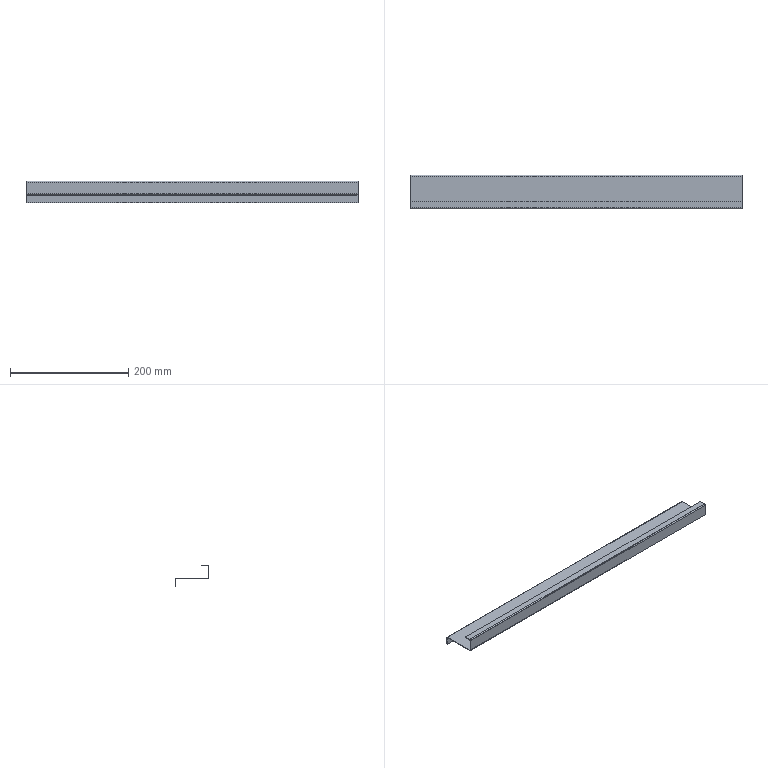Component | SolidWorks | CCQ-1.1-13UpperBeam2-1 | 1 solid | 30 faces | box 561 x 56.74 x 37 mm | volume 57303 mm3 | plane 24 | cylinder 6 | commonest cylinder face diameters 3.473 x3 1.473 x3 | material 304
STEP:
#1=COLOUR_RGB('',0.7922,0.8196,0.9333);
#2=FILL_AREA_STYLE_COLOUR('',#1);
#3=FILL_AREA_STYLE('',(#2));
#4=SURFACE_STYLE_FILL_AREA(#3);
#5=SURFACE_SIDE_STYLE('',(#4));
#6=SURFACE_STYLE_USAGE(.BOTH.,#5);
#7=PRESENTATION_STYLE_ASSIGNMENT((#6));
#8=CARTESIAN_POINT('',(-1.161,26.014,0.8164));
#9=VERTEX_POINT('',#8);
#10=CARTESIAN_POINT('',(-1.161,26.054,0.8164));
#11=VERTEX_POINT('',#10);
#12=CARTESIAN_POINT('',(-1.161,26.014,0.8164));
#13=DIRECTION('',(0.,1.,0.));
#14=VECTOR('',#13,39.37);
#15=LINE('',#12,#14);
#16=EDGE_CURVE('',#9,#11,#15,.T.);
#17=ORIENTED_EDGE('',*,*,#16,.F.);
#18=CARTESIAN_POINT('',(-1.161,26.083,0.748));
#19=VERTEX_POINT('',#18);
#20=CARTESIAN_POINT('',(-1.161,26.083,0.8164));
#21=DIRECTION('',(-1.,0.,0.));
#22=DIRECTION('',(0.,0.,-1.));
#23=AXIS2_PLACEMENT_3D('',#20,#21,#22);
#24=CIRCLE('',#23,0.06837);
#25=EDGE_CURVE('',#19,#9,#24,.T.);
#26=ORIENTED_EDGE('',*,*,#25,.F.);
#27=CARTESIAN_POINT('',(-1.161,26.083,0.7874));
#28=VERTEX_POINT('',#27);
#29=CARTESIAN_POINT('',(-1.161,26.083,0.7874));
#30=DIRECTION('',(0.,0.,-1.));
#31=VECTOR('',#30,39.37);
#32=LINE('',#29,#31);
#33=EDGE_CURVE('',#28,#19,#32,.T.);
#34=ORIENTED_EDGE('',*,*,#33,.F.);
#35=CARTESIAN_POINT('',(-1.161,26.083,0.8164));
#36=DIRECTION('',(-1.,0.,0.));
#37=DIRECTION('',(0.,0.,-1.));
#38=AXIS2_PLACEMENT_3D('',#35,#36,#37);
#39=CIRCLE('',#38,0.029);
#40=EDGE_CURVE('',#28,#11,#39,.T.);
#41=ORIENTED_EDGE('',*,*,#40,.T.);
#42=EDGE_LOOP('',(#17,#26,#34,#41));
#43=FACE_OUTER_BOUND('',#42,.T.);
#44=CARTESIAN_POINT('',(-1.161,26.014,0.8164));
#45=DIRECTION('',(1.,0.,0.));
#46=DIRECTION('',(0.,0.,-1.));
#47=AXIS2_PLACEMENT_3D('',#44,#45,#46);
#48=PLANE('',#47);
#49=ADVANCED_FACE('',(#43),#48,.T.);
#50=CARTESIAN_POINT('',(-1.161,26.014,1.585));
#51=VERTEX_POINT('',#50);
#52=CARTESIAN_POINT('',(-1.161,26.014,0.748));
#53=DIRECTION('',(0.,-0.,1.));
#54=VECTOR('',#53,39.37);
#55=LINE('',#52,#54);
#56=EDGE_CURVE('',#9,#51,#55,.T.);
#57=ORIENTED_EDGE('',*,*,#56,.F.);
#58=ORIENTED_EDGE('',*,*,#16,.T.);
#59=CARTESIAN_POINT('',(-1.161,26.054,1.585));
#60=VERTEX_POINT('',#59);
#61=CARTESIAN_POINT('',(-1.161,26.054,0.748));
#62=DIRECTION('',(0.,-0.,1.));
#63=VECTOR('',#62,39.37);
#64=LINE('',#61,#63);
#65=EDGE_CURVE('',#11,#60,#64,.T.);
#66=ORIENTED_EDGE('',*,*,#65,.T.);
#67=CARTESIAN_POINT('',(-1.161,26.054,1.585));
#68=DIRECTION('',(0.,-1.,0.));
#69=VECTOR('',#68,39.37);
#70=LINE('',#67,#69);
#71=EDGE_CURVE('',#60,#51,#70,.T.);
#72=ORIENTED_EDGE('',*,*,#71,.T.);
#73=EDGE_LOOP('',(#57,#58,#66,#72));
#74=FACE_OUTER_BOUND('',#73,.T.);
#75=CARTESIAN_POINT('',(-1.161,26.083,0.7874));
#76=DIRECTION('',(1.,0.,0.));
#77=DIRECTION('',(0.,0.,-1.));
#78=AXIS2_PLACEMENT_3D('',#75,#76,#77);
#79=PLANE('',#78);
#80=ADVANCED_FACE('',(#74),#79,.T.);
#81=CARTESIAN_POINT('',(-23.248,26.083,0.748));
#82=VERTEX_POINT('',#81);
#83=CARTESIAN_POINT('',(-23.248,26.083,0.7874));
#84=VERTEX_POINT('',#83);
#85=CARTESIAN_POINT('',(-23.248,26.083,0.748));
#86=DIRECTION('',(0.,0.,1.));
#87=VECTOR('',#86,39.37);
#88=LINE('',#85,#87);
#89=EDGE_CURVE('',#82,#84,#88,.T.);
#90=ORIENTED_EDGE('',*,*,#89,.F.);
#91=CARTESIAN_POINT('',(-23.248,26.014,0.8164));
#92=VERTEX_POINT('',#91);
#93=CARTESIAN_POINT('',(-23.248,26.083,0.8164));
#94=DIRECTION('',(-1.,0.,0.));
#95=DIRECTION('',(0.,0.,-1.));
#96=AXIS2_PLACEMENT_3D('',#93,#94,#95);
#97=CIRCLE('',#96,0.06837);
#98=EDGE_CURVE('',#82,#92,#97,.T.);
#99=ORIENTED_EDGE('',*,*,#98,.T.);
#100=CARTESIAN_POINT('',(-23.248,26.054,0.8164));
#101=VERTEX_POINT('',#100);
#102=CARTESIAN_POINT('',(-23.248,26.054,0.8164));
#103=DIRECTION('',(0.,-1.,-0.));
#104=VECTOR('',#103,39.37);
#105=LINE('',#102,#104);
#106=EDGE_CURVE('',#101,#92,#105,.T.);
#107=ORIENTED_EDGE('',*,*,#106,.F.);
#108=CARTESIAN_POINT('',(-23.248,26.083,0.8164));
#109=DIRECTION('',(-1.,0.,0.));
#110=DIRECTION('',(0.,0.,-1.));
#111=AXIS2_PLACEMENT_3D('',#108,#109,#110);
#112=CIRCLE('',#111,0.029);
#113=EDGE_CURVE('',#84,#101,#112,.T.);
#114=ORIENTED_EDGE('',*,*,#113,.F.);
#115=EDGE_LOOP('',(#90,#99,#107,#114));
#116=FACE_OUTER_BOUND('',#115,.T.);
#117=CARTESIAN_POINT('',(-23.248,26.083,0.748));
#118=DIRECTION('',(-1.,0.,0.));
#119=DIRECTION('',(0.,0.,1.));
#120=AXIS2_PLACEMENT_3D('',#117,#118,#119);
#121=PLANE('',#120);
#122=ADVANCED_FACE('',(#116),#121,.T.);
#123=CARTESIAN_POINT('',(-23.248,28.18,0.748));
#124=VERTEX_POINT('',#123);
#125=CARTESIAN_POINT('',(-23.248,28.18,0.748));
#126=DIRECTION('',(0.,-1.,0.));
#127=VECTOR('',#126,39.37);
#128=LINE('',#125,#127);
#129=EDGE_CURVE('',#124,#82,#128,.T.);
#130=ORIENTED_EDGE('',*,*,#129,.T.);
#131=ORIENTED_EDGE('',*,*,#89,.T.);
#132=CARTESIAN_POINT('',(-23.248,28.18,0.7874));
#133=VERTEX_POINT('',#132);
#134=CARTESIAN_POINT('',(-23.248,28.18,0.7874));
#135=DIRECTION('',(0.,-1.,0.));
#136=VECTOR('',#135,39.37);
#137=LINE('',#134,#136);
#138=EDGE_CURVE('',#133,#84,#137,.T.);
#139=ORIENTED_EDGE('',*,*,#138,.F.);
#140=CARTESIAN_POINT('',(-23.248,28.18,0.7874));
#141=DIRECTION('',(0.,0.,-1.));
#142=VECTOR('',#141,39.37);
#143=LINE('',#140,#142);
#144=EDGE_CURVE('',#133,#124,#143,.T.);
#145=ORIENTED_EDGE('',*,*,#144,.T.);
#146=EDGE_LOOP('',(#130,#131,#139,#145));
#147=FACE_OUTER_BOUND('',#146,.T.);
#148=CARTESIAN_POINT('',(-23.248,26.054,0.8164));
#149=DIRECTION('',(-1.,0.,0.));
#150=DIRECTION('',(0.,0.,1.));
#151=AXIS2_PLACEMENT_3D('',#148,#149,#150);
#152=PLANE('',#151);
#153=ADVANCED_FACE('',(#147),#152,.T.);
#154=CARTESIAN_POINT('',(-1.161,26.083,1.654));
#155=VERTEX_POINT('',#154);
#156=CARTESIAN_POINT('',(-1.161,26.083,1.614));
#157=VERTEX_POINT('',#156);
#158=CARTESIAN_POINT('',(-1.161,26.083,1.654));
#159=DIRECTION('',(0.,0.,-1.));
#160=VECTOR('',#159,39.37);
#161=LINE('',#158,#160);
#162=EDGE_CURVE('',#155,#157,#161,.T.);
#163=ORIENTED_EDGE('',*,*,#162,.F.);
#164=CARTESIAN_POINT('',(-1.161,26.083,1.585));
#165=DIRECTION('',(-1.,0.,0.));
#166=DIRECTION('',(0.,0.,-1.));
#167=AXIS2_PLACEMENT_3D('',#164,#165,#166);
#168=CIRCLE('',#167,0.06837);
#169=EDGE_CURVE('',#51,#155,#168,.T.);
#170=ORIENTED_EDGE('',*,*,#169,.F.);
#171=ORIENTED_EDGE('',*,*,#71,.F.);
#172=CARTESIAN_POINT('',(-1.161,26.083,1.585));
#173=DIRECTION('',(-1.,0.,0.));
#174=DIRECTION('',(0.,0.,-1.));
#175=AXIS2_PLACEMENT_3D('',#172,#173,#174);
#176=CIRCLE('',#175,0.029);
#177=EDGE_CURVE('',#60,#157,#176,.T.);
#178=ORIENTED_EDGE('',*,*,#177,.T.);
#179=EDGE_LOOP('',(#163,#170,#171,#178));
#180=FACE_OUTER_BOUND('',#179,.T.);
#181=CARTESIAN_POINT('',(-1.161,26.083,1.654));
#182=DIRECTION('',(1.,0.,0.));
#183=DIRECTION('',(0.,0.,-1.));
#184=AXIS2_PLACEMENT_3D('',#181,#182,#183);
#185=PLANE('',#184);
#186=ADVANCED_FACE('',(#180),#185,.T.);
#187=CARTESIAN_POINT('',(-1.161,26.487,1.654));
#188=VERTEX_POINT('',#187);
#189=CARTESIAN_POINT('',(-1.161,26.014,1.654));
#190=DIRECTION('',(0.,1.,0.));
#191=VECTOR('',#190,39.37);
#192=LINE('',#189,#191);
#193=EDGE_CURVE('',#155,#188,#192,.T.);
#194=ORIENTED_EDGE('',*,*,#193,.F.);
#195=ORIENTED_EDGE('',*,*,#162,.T.);
#196=CARTESIAN_POINT('',(-1.161,26.487,1.614));
#197=VERTEX_POINT('',#196);
#198=CARTESIAN_POINT('',(-1.161,26.014,1.614));
#199=DIRECTION('',(0.,1.,0.));
#200=VECTOR('',#199,39.37);
#201=LINE('',#198,#200);
#202=EDGE_CURVE('',#157,#197,#201,.T.);
#203=ORIENTED_EDGE('',*,*,#202,.T.);
#204=CARTESIAN_POINT('',(-1.161,26.487,1.654));
#205=DIRECTION('',(0.,0.,-1.));
#206=VECTOR('',#205,39.37);
#207=LINE('',#204,#206);
#208=EDGE_CURVE('',#188,#197,#207,.T.);
#209=ORIENTED_EDGE('',*,*,#208,.F.);
#210=EDGE_LOOP('',(#194,#195,#203,#209));
#211=FACE_OUTER_BOUND('',#210,.T.);
#212=CARTESIAN_POINT('',(-1.161,26.054,1.585));
#213=DIRECTION('',(1.,0.,0.));
#214=DIRECTION('',(0.,0.,-1.));
#215=AXIS2_PLACEMENT_3D('',#212,#213,#214);
#216=PLANE('',#215);
#217=ADVANCED_FACE('',(#211),#216,.T.);
#218=CARTESIAN_POINT('',(-23.248,26.014,1.585));
#219=VERTEX_POINT('',#218);
#220=CARTESIAN_POINT('',(-23.248,26.054,1.585));
#221=VERTEX_POINT('',#220);
#222=CARTESIAN_POINT('',(-23.248,26.014,1.585));
#223=DIRECTION('',(0.,1.,0.));
#224=VECTOR('',#223,39.37);
#225=LINE('',#222,#224);
#226=EDGE_CURVE('',#219,#221,#225,.T.);
#227=ORIENTED_EDGE('',*,*,#226,.F.);
#228=CARTESIAN_POINT('',(-23.248,26.083,1.654));
#229=VERTEX_POINT('',#228);
#230=CARTESIAN_POINT('',(-23.248,26.083,1.585));
#231=DIRECTION('',(-1.,0.,0.));
#232=DIRECTION('',(0.,0.,-1.));
#233=AXIS2_PLACEMENT_3D('',#230,#231,#232);
#234=CIRCLE('',#233,0.06837);
#235=EDGE_CURVE('',#219,#229,#234,.T.);
#236=ORIENTED_EDGE('',*,*,#235,.T.);
#237=CARTESIAN_POINT('',(-23.248,26.083,1.614));
#238=VERTEX_POINT('',#237);
#239=CARTESIAN_POINT('',(-23.248,26.083,1.614));
#240=DIRECTION('',(0.,0.,1.));
#241=VECTOR('',#240,39.37);
#242=LINE('',#239,#241);
#243=EDGE_CURVE('',#238,#229,#242,.T.);
#244=ORIENTED_EDGE('',*,*,#243,.F.);
#245=CARTESIAN_POINT('',(-23.248,26.083,1.585));
#246=DIRECTION('',(-1.,0.,0.));
#247=DIRECTION('',(0.,0.,-1.));
#248=AXIS2_PLACEMENT_3D('',#245,#246,#247);
#249=CIRCLE('',#248,0.029);
#250=EDGE_CURVE('',#221,#238,#249,.T.);
#251=ORIENTED_EDGE('',*,*,#250,.F.);
#252=EDGE_LOOP('',(#227,#236,#244,#251));
#253=FACE_OUTER_BOUND('',#252,.T.);
#254=CARTESIAN_POINT('',(-23.248,26.014,1.585));
#255=DIRECTION('',(-1.,0.,0.));
#256=DIRECTION('',(0.,0.,1.));
#257=AXIS2_PLACEMENT_3D('',#254,#255,#256);
#258=PLANE('',#257);
#259=ADVANCED_FACE('',(#253),#258,.T.);
#260=CARTESIAN_POINT('',(-23.248,26.014,0.748));
#261=DIRECTION('',(0.,-0.,1.));
#262=VECTOR('',#261,39.37);
#263=LINE('',#260,#262);
#264=EDGE_CURVE('',#92,#219,#263,.T.);
#265=ORIENTED_EDGE('',*,*,#264,.T.);
#266=ORIENTED_EDGE('',*,*,#226,.T.);
#267=CARTESIAN_POINT('',(-23.248,26.054,0.748));
#268=DIRECTION('',(0.,-0.,1.));
#269=VECTOR('',#268,39.37);
#270=LINE('',#267,#269);
#271=EDGE_CURVE('',#101,#221,#270,.T.);
#272=ORIENTED_EDGE('',*,*,#271,.F.);
#273=ORIENTED_EDGE('',*,*,#106,.T.);
#274=EDGE_LOOP('',(#265,#266,#272,#273));
#275=FACE_OUTER_BOUND('',#274,.T.);
#276=CARTESIAN_POINT('',(-23.248,26.083,1.614));
#277=DIRECTION('',(-1.,0.,0.));
#278=DIRECTION('',(0.,0.,1.));
#279=AXIS2_PLACEMENT_3D('',#276,#277,#278);
#280=PLANE('',#279);
#281=ADVANCED_FACE('',(#275),#280,.T.);
#282=CARTESIAN_POINT('',(-23.248,26.487,1.614));
#283=VERTEX_POINT('',#282);
#284=CARTESIAN_POINT('',(-23.248,26.014,1.614));
#285=DIRECTION('',(0.,1.,0.));
#286=VECTOR('',#285,39.37);
#287=LINE('',#284,#286);
#288=EDGE_CURVE('',#238,#283,#287,.T.);
#289=ORIENTED_EDGE('',*,*,#288,.T.);
#290=CARTESIAN_POINT('',(-1.161,26.487,1.614));
#291=DIRECTION('',(-1.,0.,0.));
#292=VECTOR('',#291,39.37);
#293=LINE('',#290,#292);
#294=EDGE_CURVE('',#197,#283,#293,.T.);
#295=ORIENTED_EDGE('',*,*,#294,.F.);
#296=ORIENTED_EDGE('',*,*,#202,.F.);
#297=CARTESIAN_POINT('',(-1.161,26.083,1.614));
#298=DIRECTION('',(-1.,0.,0.));
#299=VECTOR('',#298,39.37);
#300=LINE('',#297,#299);
#301=EDGE_CURVE('',#157,#238,#300,.T.);
#302=ORIENTED_EDGE('',*,*,#301,.T.);
#303=EDGE_LOOP('',(#289,#295,#296,#302));
#304=FACE_OUTER_BOUND('',#303,.T.);
#305=CARTESIAN_POINT('',(-1.161,26.014,1.614));
#306=DIRECTION('',(0.,0.,1.));
#307=DIRECTION('',(1.,0.,0.));
#308=AXIS2_PLACEMENT_3D('',#305,#306,#307);
#309=PLANE('',#308);
#310=ADVANCED_FACE('',(#304),#309,.F.);
#311=CARTESIAN_POINT('',(-23.248,26.487,1.654));
#312=VERTEX_POINT('',#311);
#313=CARTESIAN_POINT('',(-23.248,26.487,1.654));
#314=DIRECTION('',(0.,0.,-1.));
#315=VECTOR('',#314,39.37);
#316=LINE('',#313,#315);
#317=EDGE_CURVE('',#312,#283,#316,.T.);
#318=ORIENTED_EDGE('',*,*,#317,.F.);
#319=CARTESIAN_POINT('',(-1.161,26.487,1.654));
#320=DIRECTION('',(-1.,0.,0.));
#321=VECTOR('',#320,39.37);
#322=LINE('',#319,#321);
#323=EDGE_CURVE('',#188,#312,#322,.T.);
#324=ORIENTED_EDGE('',*,*,#323,.F.);
#325=ORIENTED_EDGE('',*,*,#208,.T.);
#326=ORIENTED_EDGE('',*,*,#294,.T.);
#327=EDGE_LOOP('',(#318,#324,#325,#326));
#328=FACE_OUTER_BOUND('',#327,.T.);
#329=CARTESIAN_POINT('',(-1.161,26.487,1.654));
#330=DIRECTION('',(0.,1.,0.));
#331=DIRECTION('',(0.,0.,1.));
#332=AXIS2_PLACEMENT_3D('',#329,#330,#331);
#333=PLANE('',#332);
#334=ADVANCED_FACE('',(#328),#333,.T.);
#335=CARTESIAN_POINT('',(-23.248,26.014,1.654));
#336=DIRECTION('',(0.,1.,0.));
#337=VECTOR('',#336,39.37);
#338=LINE('',#335,#337);
#339=EDGE_CURVE('',#229,#312,#338,.T.);
#340=ORIENTED_EDGE('',*,*,#339,.F.);
#341=CARTESIAN_POINT('',(-1.161,26.083,1.654));
#342=DIRECTION('',(-1.,0.,0.));
#343=VECTOR('',#342,39.37);
#344=LINE('',#341,#343);
#345=EDGE_CURVE('',#155,#229,#344,.T.);
#346=ORIENTED_EDGE('',*,*,#345,.F.);
#347=ORIENTED_EDGE('',*,*,#193,.T.);
#348=ORIENTED_EDGE('',*,*,#323,.T.);
#349=EDGE_LOOP('',(#340,#346,#347,#348));
#350=FACE_OUTER_BOUND('',#349,.T.);
#351=CARTESIAN_POINT('',(-1.161,26.014,1.654));
#352=DIRECTION('',(0.,0.,1.));
#353=DIRECTION('',(1.,0.,0.));
#354=AXIS2_PLACEMENT_3D('',#351,#352,#353);
#355=PLANE('',#354);
#356=ADVANCED_FACE('',(#350),#355,.T.);
#357=ORIENTED_EDGE('',*,*,#235,.F.);
#358=CARTESIAN_POINT('',(-1.161,26.014,1.585));
#359=DIRECTION('',(-1.,0.,0.));
#360=VECTOR('',#359,39.37);
#361=LINE('',#358,#360);
#362=EDGE_CURVE('',#51,#219,#361,.T.);
#363=ORIENTED_EDGE('',*,*,#362,.F.);
#364=ORIENTED_EDGE('',*,*,#169,.T.);
#365=ORIENTED_EDGE('',*,*,#345,.T.);
#366=EDGE_LOOP('',(#357,#363,#364,#365));
#367=FACE_OUTER_BOUND('',#366,.T.);
#368=CARTESIAN_POINT('',(-1.161,26.083,1.585));
#369=DIRECTION('',(-1.,0.,0.));
#370=DIRECTION('',(0.,0.,1.));
#371=AXIS2_PLACEMENT_3D('',#368,#369,#370);
#372=CYLINDRICAL_SURFACE('',#371,0.06837);
#373=ADVANCED_FACE('',(#367),#372,.T.);
#374=ORIENTED_EDGE('',*,*,#264,.F.);
#375=CARTESIAN_POINT('',(-1.161,26.014,0.8164));
#376=DIRECTION('',(-1.,0.,0.));
#377=VECTOR('',#376,39.37);
#378=LINE('',#375,#377);
#379=EDGE_CURVE('',#9,#92,#378,.T.);
#380=ORIENTED_EDGE('',*,*,#379,.F.);
#381=ORIENTED_EDGE('',*,*,#56,.T.);
#382=ORIENTED_EDGE('',*,*,#362,.T.);
#383=EDGE_LOOP('',(#374,#380,#381,#382));
#384=FACE_OUTER_BOUND('',#383,.T.);
#385=CARTESIAN_POINT('',(-1.161,26.014,0.748));
#386=DIRECTION('',(0.,-1.,-0.));
#387=DIRECTION('',(0.,0.,-1.));
#388=AXIS2_PLACEMENT_3D('',#385,#386,#387);
#389=PLANE('',#388);
#390=ADVANCED_FACE('',(#384),#389,.T.);
#391=ORIENTED_EDGE('',*,*,#98,.F.);
#392=CARTESIAN_POINT('',(-1.161,26.083,0.748));
#393=DIRECTION('',(-1.,0.,0.));
#394=VECTOR('',#393,39.37);
#395=LINE('',#392,#394);
#396=EDGE_CURVE('',#19,#82,#395,.T.);
#397=ORIENTED_EDGE('',*,*,#396,.F.);
#398=ORIENTED_EDGE('',*,*,#25,.T.);
#399=ORIENTED_EDGE('',*,*,#379,.T.);
#400=EDGE_LOOP('',(#391,#397,#398,#399));
#401=FACE_OUTER_BOUND('',#400,.T.);
#402=CARTESIAN_POINT('',(-1.161,26.083,0.8164));
#403=DIRECTION('',(-1.,0.,0.));
#404=DIRECTION('',(0.,0.,1.));
#405=AXIS2_PLACEMENT_3D('',#402,#403,#404);
#406=CYLINDRICAL_SURFACE('',#405,0.06837);
#407=ADVANCED_FACE('',(#401),#406,.T.);
#408=ORIENTED_EDGE('',*,*,#129,.F.);
#409=CARTESIAN_POINT('',(-1.161,28.18,0.748));
#410=VERTEX_POINT('',#409);
#411=CARTESIAN_POINT('',(-1.161,28.18,0.748));
#412=DIRECTION('',(-1.,0.,0.));
#413=VECTOR('',#412,39.37);
#414=LINE('',#411,#413);
#415=EDGE_CURVE('',#410,#124,#414,.T.);
#416=ORIENTED_EDGE('',*,*,#415,.F.);
#417=CARTESIAN_POINT('',(-1.161,28.18,0.748));
#418=DIRECTION('',(0.,-1.,0.));
#419=VECTOR('',#418,39.37);
#420=LINE('',#417,#419);
#421=EDGE_CURVE('',#410,#19,#420,.T.);
#422=ORIENTED_EDGE('',*,*,#421,.T.);
#423=ORIENTED_EDGE('',*,*,#396,.T.);
#424=EDGE_LOOP('',(#408,#416,#422,#423));
#425=FACE_OUTER_BOUND('',#424,.T.);
#426=CARTESIAN_POINT('',(-1.161,28.18,0.748));
#427=DIRECTION('',(0.,-0.,-1.));
#428=DIRECTION('',(0.,1.,-0.));
#429=AXIS2_PLACEMENT_3D('',#426,#427,#428);
#430=PLANE('',#429);
#431=ADVANCED_FACE('',(#425),#430,.T.);
#432=ORIENTED_EDGE('',*,*,#138,.T.);
#433=CARTESIAN_POINT('',(-1.161,26.083,0.7874));
#434=DIRECTION('',(-1.,0.,0.));
#435=VECTOR('',#434,39.37);
#436=LINE('',#433,#435);
#437=EDGE_CURVE('',#28,#84,#436,.T.);
#438=ORIENTED_EDGE('',*,*,#437,.F.);
#439=CARTESIAN_POINT('',(-1.161,28.18,0.7874));
#440=VERTEX_POINT('',#439);
#441=CARTESIAN_POINT('',(-1.161,28.18,0.7874));
#442=DIRECTION('',(0.,-1.,0.));
#443=VECTOR('',#442,39.37);
#444=LINE('',#441,#443);
#445=EDGE_CURVE('',#440,#28,#444,.T.);
#446=ORIENTED_EDGE('',*,*,#445,.F.);
#447=CARTESIAN_POINT('',(-1.161,28.18,0.7874));
#448=DIRECTION('',(-1.,0.,0.));
#449=VECTOR('',#448,39.37);
#450=LINE('',#447,#449);
#451=EDGE_CURVE('',#440,#133,#450,.T.);
#452=ORIENTED_EDGE('',*,*,#451,.T.);
#453=EDGE_LOOP('',(#432,#438,#446,#452));
#454=FACE_OUTER_BOUND('',#453,.T.);
#455=CARTESIAN_POINT('',(-1.161,28.18,0.7874));
#456=DIRECTION('',(0.,-0.,-1.));
#457=DIRECTION('',(0.,1.,-0.));
#458=AXIS2_PLACEMENT_3D('',#455,#456,#457);
#459=PLANE('',#458);
#460=ADVANCED_FACE('',(#454),#459,.F.);
#461=ORIENTED_EDGE('',*,*,#113,.T.);
#462=CARTESIAN_POINT('',(-1.161,26.054,0.8164));
#463=DIRECTION('',(-1.,0.,0.));
#464=VECTOR('',#463,39.37);
#465=LINE('',#462,#464);
#466=EDGE_CURVE('',#11,#101,#465,.T.);
#467=ORIENTED_EDGE('',*,*,#466,.F.);
#468=ORIENTED_EDGE('',*,*,#40,.F.);
#469=ORIENTED_EDGE('',*,*,#437,.T.);
#470=EDGE_LOOP('',(#461,#467,#468,#469));
#471=FACE_OUTER_BOUND('',#470,.T.);
#472=CARTESIAN_POINT('',(-1.161,26.083,0.8164));
#473=DIRECTION('',(-1.,0.,0.));
#474=DIRECTION('',(0.,0.,1.));
#475=AXIS2_PLACEMENT_3D('',#472,#473,#474);
#476=CYLINDRICAL_SURFACE('',#475,0.029);
#477=ADVANCED_FACE('',(#471),#476,.F.);
#478=ORIENTED_EDGE('',*,*,#271,.T.);
#479=CARTESIAN_POINT('',(-1.161,26.054,1.585));
#480=DIRECTION('',(-1.,0.,0.));
#481=VECTOR('',#480,39.37);
#482=LINE('',#479,#481);
#483=EDGE_CURVE('',#60,#221,#482,.T.);
#484=ORIENTED_EDGE('',*,*,#483,.F.);
#485=ORIENTED_EDGE('',*,*,#65,.F.);
#486=ORIENTED_EDGE('',*,*,#466,.T.);
#487=EDGE_LOOP('',(#478,#484,#485,#486));
#488=FACE_OUTER_BOUND('',#487,.T.);
#489=CARTESIAN_POINT('',(-1.161,26.054,0.748));
#490=DIRECTION('',(0.,-1.,-0.));
#491=DIRECTION('',(0.,0.,-1.));
#492=AXIS2_PLACEMENT_3D('',#489,#490,#491);
#493=PLANE('',#492);
#494=ADVANCED_FACE('',(#488),#493,.F.);
#495=ORIENTED_EDGE('',*,*,#250,.T.);
#496=ORIENTED_EDGE('',*,*,#301,.F.);
#497=ORIENTED_EDGE('',*,*,#177,.F.);
#498=ORIENTED_EDGE('',*,*,#483,.T.);
#499=EDGE_LOOP('',(#495,#496,#497,#498));
#500=FACE_OUTER_BOUND('',#499,.T.);
#501=CARTESIAN_POINT('',(-1.161,26.083,1.585));
#502=DIRECTION('',(-1.,0.,0.));
#503=DIRECTION('',(0.,0.,1.));
#504=AXIS2_PLACEMENT_3D('',#501,#502,#503);
#505=CYLINDRICAL_SURFACE('',#504,0.029);
#506=ADVANCED_FACE('',(#500),#505,.F.);
#507=ORIENTED_EDGE('',*,*,#445,.T.);
#508=ORIENTED_EDGE('',*,*,#33,.T.);
#509=ORIENTED_EDGE('',*,*,#421,.F.);
#510=CARTESIAN_POINT('',(-1.161,28.18,0.7874));
#511=DIRECTION('',(0.,0.,-1.));
#512=VECTOR('',#511,39.37);
#513=LINE('',#510,#512);
#514=EDGE_CURVE('',#440,#410,#513,.T.);
#515=ORIENTED_EDGE('',*,*,#514,.F.);
#516=EDGE_LOOP('',(#507,#508,#509,#515));
#517=FACE_OUTER_BOUND('',#516,.T.);
#518=CARTESIAN_POINT('',(-1.161,26.083,1.585));
#519=DIRECTION('',(1.,0.,0.));
#520=DIRECTION('',(0.,0.,-1.));
#521=AXIS2_PLACEMENT_3D('',#518,#519,#520);
#522=PLANE('',#521);
#523=ADVANCED_FACE('',(#517),#522,.T.);
#524=ORIENTED_EDGE('',*,*,#288,.F.);
#525=ORIENTED_EDGE('',*,*,#243,.T.);
#526=ORIENTED_EDGE('',*,*,#339,.T.);
#527=ORIENTED_EDGE('',*,*,#317,.T.);
#528=EDGE_LOOP('',(#524,#525,#526,#527));
#529=FACE_OUTER_BOUND('',#528,.T.);
#530=CARTESIAN_POINT('',(-23.248,26.083,1.585));
#531=DIRECTION('',(1.,0.,0.));
#532=DIRECTION('',(0.,0.,-1.));
#533=AXIS2_PLACEMENT_3D('',#530,#531,#532);
#534=PLANE('',#533);
#535=ADVANCED_FACE('',(#529),#534,.F.);
#536=CARTESIAN_POINT('',(-23.248,28.209,0.719));
#537=VERTEX_POINT('',#536);
#538=CARTESIAN_POINT('',(-23.248,28.248,0.719));
#539=VERTEX_POINT('',#538);
#540=CARTESIAN_POINT('',(-23.248,28.248,0.719));
#541=DIRECTION('',(-0.,1.,0.));
#542=VECTOR('',#541,39.37);
#543=LINE('',#540,#542);
#544=EDGE_CURVE('',#537,#539,#543,.T.);
#545=ORIENTED_EDGE('',*,*,#544,.F.);
#546=CARTESIAN_POINT('',(-23.248,28.18,0.719));
#547=DIRECTION('',(-1.,0.,0.));
#548=DIRECTION('',(0.,0.,-1.));
#549=AXIS2_PLACEMENT_3D('',#546,#547,#548);
#550=CIRCLE('',#549,0.029);
#551=EDGE_CURVE('',#124,#537,#550,.T.);
#552=ORIENTED_EDGE('',*,*,#551,.F.);
#553=ORIENTED_EDGE('',*,*,#144,.F.);
#554=CARTESIAN_POINT('',(-23.248,28.18,0.719));
#555=DIRECTION('',(-1.,0.,0.));
#556=DIRECTION('',(0.,0.,-1.));
#557=AXIS2_PLACEMENT_3D('',#554,#555,#556);
#558=CIRCLE('',#557,0.06837);
#559=EDGE_CURVE('',#133,#539,#558,.T.);
#560=ORIENTED_EDGE('',*,*,#559,.T.);
#561=EDGE_LOOP('',(#545,#552,#553,#560));
#562=FACE_OUTER_BOUND('',#561,.T.);
#563=CARTESIAN_POINT('',(-23.248,28.18,0.719));
#564=DIRECTION('',(-1.,0.,0.));
#565=DIRECTION('',(0.,0.,1.));
#566=AXIS2_PLACEMENT_3D('',#563,#564,#565);
#567=PLANE('',#566);
#568=ADVANCED_FACE('',(#562),#567,.T.);
#569=CARTESIAN_POINT('',(-1.161,28.209,0.719));
#570=VERTEX_POINT('',#569);
#571=CARTESIAN_POINT('',(-1.161,28.18,0.719));
#572=DIRECTION('',(1.,0.,0.));
#573=DIRECTION('',(0.,0.,-1.));
#574=AXIS2_PLACEMENT_3D('',#571,#572,#573);
#575=CIRCLE('',#574,0.029);
#576=EDGE_CURVE('',#570,#410,#575,.T.);
#577=ORIENTED_EDGE('',*,*,#576,.F.);
#578=CARTESIAN_POINT('',(-1.161,28.248,0.719));
#579=VERTEX_POINT('',#578);
#580=CARTESIAN_POINT('',(-1.161,28.209,0.719));
#581=DIRECTION('',(0.,1.,0.));
#582=VECTOR('',#581,39.37);
#583=LINE('',#580,#582);
#584=EDGE_CURVE('',#570,#579,#583,.T.);
#585=ORIENTED_EDGE('',*,*,#584,.T.);
#586=CARTESIAN_POINT('',(-1.161,28.18,0.719));
#587=DIRECTION('',(1.,0.,0.));
#588=DIRECTION('',(0.,0.,-1.));
#589=AXIS2_PLACEMENT_3D('',#586,#587,#588);
#590=CIRCLE('',#589,0.06837);
#591=EDGE_CURVE('',#579,#440,#590,.T.);
#592=ORIENTED_EDGE('',*,*,#591,.T.);
#593=ORIENTED_EDGE('',*,*,#514,.T.);
#594=EDGE_LOOP('',(#577,#585,#592,#593));
#595=FACE_OUTER_BOUND('',#594,.T.);
#596=CARTESIAN_POINT('',(-1.161,28.18,0.719));
#597=DIRECTION('',(-1.,0.,0.));
#598=DIRECTION('',(0.,0.,1.));
#599=AXIS2_PLACEMENT_3D('',#596,#597,#598);
#600=PLANE('',#599);
#601=ADVANCED_FACE('',(#595),#600,.F.);
#602=ORIENTED_EDGE('',*,*,#451,.F.);
#603=ORIENTED_EDGE('',*,*,#591,.F.);
#604=CARTESIAN_POINT('',(-12.205,28.248,0.719));
#605=DIRECTION('',(1.,-0.,0.));
#606=VECTOR('',#605,39.37);
#607=LINE('',#604,#606);
#608=EDGE_CURVE('',#539,#579,#607,.T.);
#609=ORIENTED_EDGE('',*,*,#608,.F.);
#610=ORIENTED_EDGE('',*,*,#559,.F.);
#611=EDGE_LOOP('',(#602,#603,#609,#610));
#612=FACE_OUTER_BOUND('',#611,.T.);
#613=CARTESIAN_POINT('',(-1.161,28.18,0.719));
#614=DIRECTION('',(1.,0.,0.));
#615=DIRECTION('',(0.,1.,0.));
#616=AXIS2_PLACEMENT_3D('',#613,#614,#615);
#617=CYLINDRICAL_SURFACE('',#616,0.06837);
#618=ADVANCED_FACE('',(#612),#617,.T.);
#619=ORIENTED_EDGE('',*,*,#415,.T.);
#620=ORIENTED_EDGE('',*,*,#551,.T.);
#621=CARTESIAN_POINT('',(-23.248,28.209,0.719));
#622=DIRECTION('',(1.,-0.,0.));
#623=VECTOR('',#622,39.37);
#624=LINE('',#621,#623);
#625=EDGE_CURVE('',#537,#570,#624,.T.);
#626=ORIENTED_EDGE('',*,*,#625,.T.);
#627=ORIENTED_EDGE('',*,*,#576,.T.);
#628=EDGE_LOOP('',(#619,#620,#626,#627));
#629=FACE_OUTER_BOUND('',#628,.T.);
#630=CARTESIAN_POINT('',(-1.161,28.18,0.719));
#631=DIRECTION('',(1.,0.,0.));
#632=DIRECTION('',(0.,1.,0.));
#633=AXIS2_PLACEMENT_3D('',#630,#631,#632);
#634=CYLINDRICAL_SURFACE('',#633,0.029);
#635=ADVANCED_FACE('',(#629),#634,.F.);
#636=CARTESIAN_POINT('',(-1.161,28.248,0.1969));
#637=VERTEX_POINT('',#636);
#638=CARTESIAN_POINT('',(-1.161,28.248,0.748));
#639=DIRECTION('',(-0.,-0.,1.));
#640=VECTOR('',#639,39.37);
#641=LINE('',#638,#640);
#642=EDGE_CURVE('',#637,#579,#641,.T.);
#643=ORIENTED_EDGE('',*,*,#642,.T.);
#644=ORIENTED_EDGE('',*,*,#584,.F.);
#645=CARTESIAN_POINT('',(-1.161,28.209,0.1969));
#646=VERTEX_POINT('',#645);
#647=CARTESIAN_POINT('',(-1.161,28.209,0.748));
#648=DIRECTION('',(-0.,-0.,1.));
#649=VECTOR('',#648,39.37);
#650=LINE('',#647,#649);
#651=EDGE_CURVE('',#646,#570,#650,.T.);
#652=ORIENTED_EDGE('',*,*,#651,.F.);
#653=CARTESIAN_POINT('',(-1.161,28.248,0.1969));
#654=DIRECTION('',(0.,-1.,-0.));
#655=VECTOR('',#654,39.37);
#656=LINE('',#653,#655);
#657=EDGE_CURVE('',#637,#646,#656,.T.);
#658=ORIENTED_EDGE('',*,*,#657,.F.);
#659=EDGE_LOOP('',(#643,#644,#652,#658));
#660=FACE_OUTER_BOUND('',#659,.T.);
#661=CARTESIAN_POINT('',(-1.161,28.248,0.748));
#662=DIRECTION('',(1.,-0.,0.));
#663=DIRECTION('',(0.,0.,-1.));
#664=AXIS2_PLACEMENT_3D('',#661,#662,#663);
#665=PLANE('',#664);
#666=ADVANCED_FACE('',(#660),#665,.T.);
#667=CARTESIAN_POINT('',(-23.248,28.209,0.1969));
#668=VERTEX_POINT('',#667);
#669=CARTESIAN_POINT('',(-23.248,28.209,0.748));
#670=DIRECTION('',(-0.,0.,-1.));
#671=VECTOR('',#670,39.37);
#672=LINE('',#669,#671);
#673=EDGE_CURVE('',#537,#668,#672,.T.);
#674=ORIENTED_EDGE('',*,*,#673,.F.);
#675=ORIENTED_EDGE('',*,*,#544,.T.);
#676=CARTESIAN_POINT('',(-23.248,28.248,0.1969));
#677=VERTEX_POINT('',#676);
#678=CARTESIAN_POINT('',(-23.248,28.248,0.1969));
#679=DIRECTION('',(-0.,0.,-1.));
#680=VECTOR('',#679,39.37);
#681=LINE('',#678,#680);
#682=EDGE_CURVE('',#539,#677,#681,.T.);
#683=ORIENTED_EDGE('',*,*,#682,.T.);
#684=CARTESIAN_POINT('',(-23.248,28.248,0.1969));
#685=DIRECTION('',(0.,-1.,-0.));
#686=VECTOR('',#685,39.37);
#687=LINE('',#684,#686);
#688=EDGE_CURVE('',#677,#668,#687,.T.);
#689=ORIENTED_EDGE('',*,*,#688,.T.);
#690=EDGE_LOOP('',(#674,#675,#683,#689));
#691=FACE_OUTER_BOUND('',#690,.T.);
#692=CARTESIAN_POINT('',(-23.248,28.248,0.1969));
#693=DIRECTION('',(-1.,-0.,0.));
#694=DIRECTION('',(0.,0.,1.));
#695=AXIS2_PLACEMENT_3D('',#692,#693,#694);
#696=PLANE('',#695);
#697=ADVANCED_FACE('',(#691),#696,.T.);
#698=ORIENTED_EDGE('',*,*,#682,.F.);
#699=ORIENTED_EDGE('',*,*,#608,.T.);
#700=ORIENTED_EDGE('',*,*,#642,.F.);
#701=CARTESIAN_POINT('',(-1.161,28.248,0.1969));
#702=DIRECTION('',(1.,0.,0.));
#703=VECTOR('',#702,39.37);
#704=LINE('',#701,#703);
#705=EDGE_CURVE('',#677,#637,#704,.T.);
#706=ORIENTED_EDGE('',*,*,#705,.F.);
#707=EDGE_LOOP('',(#698,#699,#700,#706));
#708=FACE_OUTER_BOUND('',#707,.T.);
#709=CARTESIAN_POINT('',(-12.205,28.248,0.748));
#710=DIRECTION('',(0.,1.,0.));
#711=DIRECTION('',(0.,-0.,1.));
#712=AXIS2_PLACEMENT_3D('',#709,#710,#711);
#713=PLANE('',#712);
#714=ADVANCED_FACE('',(#708),#713,.T.);
#715=ORIENTED_EDGE('',*,*,#625,.F.);
#716=ORIENTED_EDGE('',*,*,#673,.T.);
#717=CARTESIAN_POINT('',(-12.205,28.209,0.1969));
#718=DIRECTION('',(1.,0.,0.));
#719=VECTOR('',#718,39.37);
#720=LINE('',#717,#719);
#721=EDGE_CURVE('',#668,#646,#720,.T.);
#722=ORIENTED_EDGE('',*,*,#721,.T.);
#723=ORIENTED_EDGE('',*,*,#651,.T.);
#724=EDGE_LOOP('',(#715,#716,#722,#723));
#725=FACE_OUTER_BOUND('',#724,.T.);
#726=CARTESIAN_POINT('',(-12.205,28.209,0.748));
#727=DIRECTION('',(0.,1.,0.));
#728=DIRECTION('',(0.,-0.,1.));
#729=AXIS2_PLACEMENT_3D('',#726,#727,#728);
#730=PLANE('',#729);
#731=ADVANCED_FACE('',(#725),#730,.F.);
#732=ORIENTED_EDGE('',*,*,#721,.F.);
#733=ORIENTED_EDGE('',*,*,#688,.F.);
#734=ORIENTED_EDGE('',*,*,#705,.T.);
#735=ORIENTED_EDGE('',*,*,#657,.T.);
#736=EDGE_LOOP('',(#732,#733,#734,#735));
#737=FACE_OUTER_BOUND('',#736,.T.);
#738=CARTESIAN_POINT('',(-1.161,28.248,0.1969));
#739=DIRECTION('',(0.,0.,-1.));
#740=DIRECTION('',(0.,1.,0.));
#741=AXIS2_PLACEMENT_3D('',#738,#739,#740);
#742=PLANE('',#741);
#743=ADVANCED_FACE('',(#737),#742,.T.);
#744=CLOSED_SHELL('',(#49,#80,#122,#153,#186,#217,#259,#281,#310,#334,#356,#373,#390,#407,#431,#460,#477,#494,#506,#523,#535,#568,#601,#618,#635,#666,#697,#714,#731,#743));
#745=MANIFOLD_SOLID_BREP('',#744);
#746=STYLED_ITEM('',(#7),#745);
#747=(LENGTH_UNIT()NAMED_UNIT(*)SI_UNIT($,.METRE.));
#748=LENGTH_MEASURE_WITH_UNIT(LENGTH_MEASURE(0.0254),#747);
#749=DIMENSIONAL_EXPONENTS(1.,0.,0.,0.,0.,0.,0.);
#750=(CONVERSION_BASED_UNIT('',#748)LENGTH_UNIT()NAMED_UNIT(#749));
#751=UNCERTAINTY_MEASURE_WITH_UNIT(LENGTH_MEASURE(0.00001),#750,'','');
#752=(NAMED_UNIT(*)PLANE_ANGLE_UNIT()SI_UNIT($,.RADIAN.));
#753=(NAMED_UNIT(*)SI_UNIT($,.STERADIAN.)SOLID_ANGLE_UNIT());
#754=(GEOMETRIC_REPRESENTATION_CONTEXT(3)GLOBAL_UNCERTAINTY_ASSIGNED_CONTEXT((#751))GLOBAL_UNIT_ASSIGNED_CONTEXT((#750,#752,#753))REPRESENTATION_CONTEXT('',''));
#755=MECHANICAL_DESIGN_GEOMETRIC_PRESENTATION_REPRESENTATION('',(#746),#754);
#756=PRESENTATION_LAYER_ASSIGNMENT('','',(#746));
#757=CARTESIAN_POINT('',(0.,0.,0.));
#758=DIRECTION('',(0.,0.,1.));
#759=DIRECTION('',(1.,0.,0.));
#760=AXIS2_PLACEMENT_3D('',#757,#758,#759);
#761=(LENGTH_UNIT()NAMED_UNIT(*)SI_UNIT($,.METRE.));
#762=LENGTH_MEASURE_WITH_UNIT(LENGTH_MEASURE(0.0254),#761);
#763=DIMENSIONAL_EXPONENTS(1.,0.,0.,0.,0.,0.,0.);
#764=(CONVERSION_BASED_UNIT('',#762)LENGTH_UNIT()NAMED_UNIT(#763));
#765=UNCERTAINTY_MEASURE_WITH_UNIT(LENGTH_MEASURE(0.00001),#764,'','');
#766=(NAMED_UNIT(*)PLANE_ANGLE_UNIT()SI_UNIT($,.RADIAN.));
#767=(NAMED_UNIT(*)SI_UNIT($,.STERADIAN.)SOLID_ANGLE_UNIT());
#768=(GEOMETRIC_REPRESENTATION_CONTEXT(3)GLOBAL_UNCERTAINTY_ASSIGNED_CONTEXT((#765))GLOBAL_UNIT_ASSIGNED_CONTEXT((#764,#766,#767))REPRESENTATION_CONTEXT('',''));
#769=ADVANCED_BREP_SHAPE_REPRESENTATION('',(#745,#760),#768);